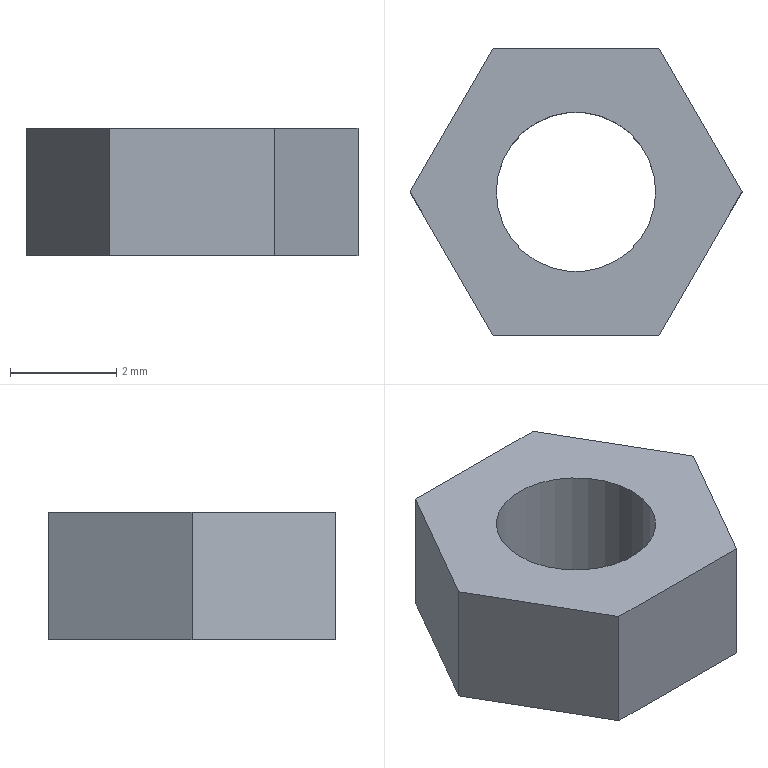Component | NX | NUT | 1 solid | 9 faces | box 6.25 x 5.41 x 2.4 mm | volume 44 mm3 | plane 8 | cylinder 1 | commonest cylinder face diameters 3 x1
STEP:
#1=CARTESIAN_POINT('',(0.,0.,0.));
#2=DIRECTION('',(0.,0.,1.));
#3=DIRECTION('',(1.,0.,0.));
#4=AXIS2_PLACEMENT_3D('',#1,#2,#3);
#5=CARTESIAN_POINT('',(-103.343,127.67,-8.98));
#6=VERTEX_POINT('',#5);
#7=CARTESIAN_POINT('',(-101.781,124.965,-8.98));
#8=VERTEX_POINT('',#7);
#9=CARTESIAN_POINT('',(-103.343,127.67,-8.98));
#10=DIRECTION('',(0.5,-0.866,0.));
#11=VECTOR('',#10,1.);
#12=LINE('',#9,#11);
#13=CARTESIAN_POINT('',(-103.343,127.67,-11.38));
#14=DIRECTION('',(-0.866,-0.5,0.));
#15=DIRECTION('',(0.5,-0.866,0.));
#16=AXIS2_PLACEMENT_3D('',#13,#14,#15);
#17=PLANE('',#16);
#18=CARTESIAN_POINT('',(0.,2.4));
#19=DIRECTION('',(1.,0.));
#20=VECTOR('',#19,1.);
#21=LINE('',#18,#20);
#22=(GEOMETRIC_REPRESENTATION_CONTEXT(2)PARAMETRIC_REPRESENTATION_CONTEXT()REPRESENTATION_CONTEXT('',''));
#23=DEFINITIONAL_REPRESENTATION('',(#21),#22);
#24=PCURVE('',#17,#23);
#25=CARTESIAN_POINT('',(-100.219,127.67,-8.98));
#26=DIRECTION('',(0.,0.,1.));
#27=DIRECTION('',(1.,0.,0.));
#28=AXIS2_PLACEMENT_3D('',#25,#26,#27);
#29=PLANE('',#28);
#30=CARTESIAN_POINT('',(-3.123,0.));
#31=DIRECTION('',(0.5,-0.866));
#32=VECTOR('',#31,1.);
#33=LINE('',#30,#32);
#34=(GEOMETRIC_REPRESENTATION_CONTEXT(2)PARAMETRIC_REPRESENTATION_CONTEXT()REPRESENTATION_CONTEXT('',''));
#35=DEFINITIONAL_REPRESENTATION('',(#33),#34);
#36=PCURVE('',#29,#35);
#37=SURFACE_CURVE('',#12,(#24,#36),.PCURVE_S1.);
#38=EDGE_CURVE('',#6,#8,#37,.T.);
#39=ORIENTED_EDGE('',*,*,#38,.F.);
#40=CARTESIAN_POINT('',(-103.343,127.67,-11.38));
#41=VERTEX_POINT('',#40);
#42=CARTESIAN_POINT('',(-103.343,127.67,-11.38));
#43=DIRECTION('',(0.,0.,1.));
#44=VECTOR('',#43,1.);
#45=LINE('',#42,#44);
#46=CARTESIAN_POINT('',(0.,0.));
#47=DIRECTION('',(0.,1.));
#48=VECTOR('',#47,1.);
#49=LINE('',#46,#48);
#50=(GEOMETRIC_REPRESENTATION_CONTEXT(2)PARAMETRIC_REPRESENTATION_CONTEXT()REPRESENTATION_CONTEXT('',''));
#51=DEFINITIONAL_REPRESENTATION('',(#49),#50);
#52=PCURVE('',#17,#51);
#53=CARTESIAN_POINT('',(-101.781,130.375,-11.38));
#54=DIRECTION('',(-0.866,0.5,0.));
#55=DIRECTION('',(-0.5,-0.866,0.));
#56=AXIS2_PLACEMENT_3D('',#53,#54,#55);
#57=PLANE('',#56);
#58=CARTESIAN_POINT('',(3.123,0.));
#59=DIRECTION('',(0.,1.));
#60=VECTOR('',#59,1.);
#61=LINE('',#58,#60);
#62=(GEOMETRIC_REPRESENTATION_CONTEXT(2)PARAMETRIC_REPRESENTATION_CONTEXT()REPRESENTATION_CONTEXT('',''));
#63=DEFINITIONAL_REPRESENTATION('',(#61),#62);
#64=PCURVE('',#57,#63);
#65=SURFACE_CURVE('',#45,(#52,#64),.PCURVE_S1.);
#66=EDGE_CURVE('',#41,#6,#65,.T.);
#67=ORIENTED_EDGE('',*,*,#66,.F.);
#68=CARTESIAN_POINT('',(-101.781,124.965,-11.38));
#69=VERTEX_POINT('',#68);
#70=CARTESIAN_POINT('',(-103.343,127.67,-11.38));
#71=DIRECTION('',(0.5,-0.866,0.));
#72=VECTOR('',#71,1.);
#73=LINE('',#70,#72);
#74=CARTESIAN_POINT('',(0.,0.));
#75=DIRECTION('',(1.,0.));
#76=VECTOR('',#75,1.);
#77=LINE('',#74,#76);
#78=(GEOMETRIC_REPRESENTATION_CONTEXT(2)PARAMETRIC_REPRESENTATION_CONTEXT()REPRESENTATION_CONTEXT('',''));
#79=DEFINITIONAL_REPRESENTATION('',(#77),#78);
#80=PCURVE('',#17,#79);
#81=CARTESIAN_POINT('',(-100.219,127.67,-11.38));
#82=DIRECTION('',(0.,0.,1.));
#83=DIRECTION('',(1.,0.,0.));
#84=AXIS2_PLACEMENT_3D('',#81,#82,#83);
#85=PLANE('',#84);
#86=CARTESIAN_POINT('',(-3.123,0.));
#87=DIRECTION('',(0.5,-0.866));
#88=VECTOR('',#87,1.);
#89=LINE('',#86,#88);
#90=(GEOMETRIC_REPRESENTATION_CONTEXT(2)PARAMETRIC_REPRESENTATION_CONTEXT()REPRESENTATION_CONTEXT('',''));
#91=DEFINITIONAL_REPRESENTATION('',(#89),#90);
#92=PCURVE('',#85,#91);
#93=SURFACE_CURVE('',#73,(#80,#92),.PCURVE_S1.);
#94=EDGE_CURVE('',#41,#69,#93,.T.);
#95=ORIENTED_EDGE('',*,*,#94,.T.);
#96=CARTESIAN_POINT('',(-101.781,124.965,-11.38));
#97=DIRECTION('',(0.,0.,1.));
#98=VECTOR('',#97,1.);
#99=LINE('',#96,#98);
#100=CARTESIAN_POINT('',(3.123,0.));
#101=DIRECTION('',(0.,1.));
#102=VECTOR('',#101,1.);
#103=LINE('',#100,#102);
#104=(GEOMETRIC_REPRESENTATION_CONTEXT(2)PARAMETRIC_REPRESENTATION_CONTEXT()REPRESENTATION_CONTEXT('',''));
#105=DEFINITIONAL_REPRESENTATION('',(#103),#104);
#106=PCURVE('',#17,#105);
#107=CARTESIAN_POINT('',(-101.781,124.965,-11.38));
#108=DIRECTION('',(-0.,-1.,0.));
#109=DIRECTION('',(1.,-0.,0.));
#110=AXIS2_PLACEMENT_3D('',#107,#108,#109);
#111=PLANE('',#110);
#112=CARTESIAN_POINT('',(0.,0.));
#113=DIRECTION('',(0.,1.));
#114=VECTOR('',#113,1.);
#115=LINE('',#112,#114);
#116=(GEOMETRIC_REPRESENTATION_CONTEXT(2)PARAMETRIC_REPRESENTATION_CONTEXT()REPRESENTATION_CONTEXT('',''));
#117=DEFINITIONAL_REPRESENTATION('',(#115),#116);
#118=PCURVE('',#111,#117);
#119=SURFACE_CURVE('',#99,(#106,#118),.PCURVE_S1.);
#120=EDGE_CURVE('',#69,#8,#119,.T.);
#121=ORIENTED_EDGE('',*,*,#120,.T.);
#122=EDGE_LOOP('',(#39,#67,#95,#121));
#123=FACE_BOUND('',#122,.T.);
#124=ADVANCED_FACE('',(#123),#17,.T.);
#125=CARTESIAN_POINT('',(-98.657,124.965,-8.98));
#126=VERTEX_POINT('',#125);
#127=CARTESIAN_POINT('',(-101.781,124.965,-8.98));
#128=DIRECTION('',(1.,-0.,0.));
#129=VECTOR('',#128,1.);
#130=LINE('',#127,#129);
#131=CARTESIAN_POINT('',(0.,2.4));
#132=DIRECTION('',(1.,0.));
#133=VECTOR('',#132,1.);
#134=LINE('',#131,#133);
#135=(GEOMETRIC_REPRESENTATION_CONTEXT(2)PARAMETRIC_REPRESENTATION_CONTEXT()REPRESENTATION_CONTEXT('',''));
#136=DEFINITIONAL_REPRESENTATION('',(#134),#135);
#137=PCURVE('',#111,#136);
#138=CARTESIAN_POINT('',(-1.562,-2.705));
#139=DIRECTION('',(1.,-0.));
#140=VECTOR('',#139,1.);
#141=LINE('',#138,#140);
#142=(GEOMETRIC_REPRESENTATION_CONTEXT(2)PARAMETRIC_REPRESENTATION_CONTEXT()REPRESENTATION_CONTEXT('',''));
#143=DEFINITIONAL_REPRESENTATION('',(#141),#142);
#144=PCURVE('',#29,#143);
#145=SURFACE_CURVE('',#130,(#137,#144),.PCURVE_S1.);
#146=EDGE_CURVE('',#8,#126,#145,.T.);
#147=ORIENTED_EDGE('',*,*,#146,.F.);
#148=ORIENTED_EDGE('',*,*,#120,.F.);
#149=CARTESIAN_POINT('',(-98.657,124.965,-11.38));
#150=VERTEX_POINT('',#149);
#151=CARTESIAN_POINT('',(-101.781,124.965,-11.38));
#152=DIRECTION('',(1.,-0.,0.));
#153=VECTOR('',#152,1.);
#154=LINE('',#151,#153);
#155=CARTESIAN_POINT('',(0.,0.));
#156=DIRECTION('',(1.,0.));
#157=VECTOR('',#156,1.);
#158=LINE('',#155,#157);
#159=(GEOMETRIC_REPRESENTATION_CONTEXT(2)PARAMETRIC_REPRESENTATION_CONTEXT()REPRESENTATION_CONTEXT('',''));
#160=DEFINITIONAL_REPRESENTATION('',(#158),#159);
#161=PCURVE('',#111,#160);
#162=CARTESIAN_POINT('',(-1.562,-2.705));
#163=DIRECTION('',(1.,-0.));
#164=VECTOR('',#163,1.);
#165=LINE('',#162,#164);
#166=(GEOMETRIC_REPRESENTATION_CONTEXT(2)PARAMETRIC_REPRESENTATION_CONTEXT()REPRESENTATION_CONTEXT('',''));
#167=DEFINITIONAL_REPRESENTATION('',(#165),#166);
#168=PCURVE('',#85,#167);
#169=SURFACE_CURVE('',#154,(#161,#168),.PCURVE_S1.);
#170=EDGE_CURVE('',#69,#150,#169,.T.);
#171=ORIENTED_EDGE('',*,*,#170,.T.);
#172=CARTESIAN_POINT('',(-98.657,124.965,-11.38));
#173=DIRECTION('',(0.,0.,1.));
#174=VECTOR('',#173,1.);
#175=LINE('',#172,#174);
#176=CARTESIAN_POINT('',(3.123,0.));
#177=DIRECTION('',(0.,1.));
#178=VECTOR('',#177,1.);
#179=LINE('',#176,#178);
#180=(GEOMETRIC_REPRESENTATION_CONTEXT(2)PARAMETRIC_REPRESENTATION_CONTEXT()REPRESENTATION_CONTEXT('',''));
#181=DEFINITIONAL_REPRESENTATION('',(#179),#180);
#182=PCURVE('',#111,#181);
#183=CARTESIAN_POINT('',(-98.657,124.965,-11.38));
#184=DIRECTION('',(0.866,-0.5,0.));
#185=DIRECTION('',(0.5,0.866,0.));
#186=AXIS2_PLACEMENT_3D('',#183,#184,#185);
#187=PLANE('',#186);
#188=CARTESIAN_POINT('',(0.,0.));
#189=DIRECTION('',(0.,1.));
#190=VECTOR('',#189,1.);
#191=LINE('',#188,#190);
#192=(GEOMETRIC_REPRESENTATION_CONTEXT(2)PARAMETRIC_REPRESENTATION_CONTEXT()REPRESENTATION_CONTEXT('',''));
#193=DEFINITIONAL_REPRESENTATION('',(#191),#192);
#194=PCURVE('',#187,#193);
#195=SURFACE_CURVE('',#175,(#182,#194),.PCURVE_S1.);
#196=EDGE_CURVE('',#150,#126,#195,.T.);
#197=ORIENTED_EDGE('',*,*,#196,.T.);
#198=EDGE_LOOP('',(#147,#148,#171,#197));
#199=FACE_BOUND('',#198,.T.);
#200=ADVANCED_FACE('',(#199),#111,.T.);
#201=CARTESIAN_POINT('',(-97.096,127.67,-8.98));
#202=VERTEX_POINT('',#201);
#203=CARTESIAN_POINT('',(-98.657,124.965,-8.98));
#204=DIRECTION('',(0.5,0.866,0.));
#205=VECTOR('',#204,1.);
#206=LINE('',#203,#205);
#207=CARTESIAN_POINT('',(0.,2.4));
#208=DIRECTION('',(1.,0.));
#209=VECTOR('',#208,1.);
#210=LINE('',#207,#209);
#211=(GEOMETRIC_REPRESENTATION_CONTEXT(2)PARAMETRIC_REPRESENTATION_CONTEXT()REPRESENTATION_CONTEXT('',''));
#212=DEFINITIONAL_REPRESENTATION('',(#210),#211);
#213=PCURVE('',#187,#212);
#214=CARTESIAN_POINT('',(1.562,-2.705));
#215=DIRECTION('',(0.5,0.866));
#216=VECTOR('',#215,1.);
#217=LINE('',#214,#216);
#218=(GEOMETRIC_REPRESENTATION_CONTEXT(2)PARAMETRIC_REPRESENTATION_CONTEXT()REPRESENTATION_CONTEXT('',''));
#219=DEFINITIONAL_REPRESENTATION('',(#217),#218);
#220=PCURVE('',#29,#219);
#221=SURFACE_CURVE('',#206,(#213,#220),.PCURVE_S1.);
#222=EDGE_CURVE('',#126,#202,#221,.T.);
#223=ORIENTED_EDGE('',*,*,#222,.F.);
#224=ORIENTED_EDGE('',*,*,#196,.F.);
#225=CARTESIAN_POINT('',(-97.096,127.67,-11.38));
#226=VERTEX_POINT('',#225);
#227=CARTESIAN_POINT('',(-98.657,124.965,-11.38));
#228=DIRECTION('',(0.5,0.866,0.));
#229=VECTOR('',#228,1.);
#230=LINE('',#227,#229);
#231=CARTESIAN_POINT('',(0.,0.));
#232=DIRECTION('',(1.,0.));
#233=VECTOR('',#232,1.);
#234=LINE('',#231,#233);
#235=(GEOMETRIC_REPRESENTATION_CONTEXT(2)PARAMETRIC_REPRESENTATION_CONTEXT()REPRESENTATION_CONTEXT('',''));
#236=DEFINITIONAL_REPRESENTATION('',(#234),#235);
#237=PCURVE('',#187,#236);
#238=CARTESIAN_POINT('',(1.562,-2.705));
#239=DIRECTION('',(0.5,0.866));
#240=VECTOR('',#239,1.);
#241=LINE('',#238,#240);
#242=(GEOMETRIC_REPRESENTATION_CONTEXT(2)PARAMETRIC_REPRESENTATION_CONTEXT()REPRESENTATION_CONTEXT('',''));
#243=DEFINITIONAL_REPRESENTATION('',(#241),#242);
#244=PCURVE('',#85,#243);
#245=SURFACE_CURVE('',#230,(#237,#244),.PCURVE_S1.);
#246=EDGE_CURVE('',#150,#226,#245,.T.);
#247=ORIENTED_EDGE('',*,*,#246,.T.);
#248=CARTESIAN_POINT('',(-97.096,127.67,-11.38));
#249=DIRECTION('',(0.,0.,1.));
#250=VECTOR('',#249,1.);
#251=LINE('',#248,#250);
#252=CARTESIAN_POINT('',(3.123,0.));
#253=DIRECTION('',(0.,1.));
#254=VECTOR('',#253,1.);
#255=LINE('',#252,#254);
#256=(GEOMETRIC_REPRESENTATION_CONTEXT(2)PARAMETRIC_REPRESENTATION_CONTEXT()REPRESENTATION_CONTEXT('',''));
#257=DEFINITIONAL_REPRESENTATION('',(#255),#256);
#258=PCURVE('',#187,#257);
#259=CARTESIAN_POINT('',(-97.096,127.67,-11.38));
#260=DIRECTION('',(0.866,0.5,0.));
#261=DIRECTION('',(-0.5,0.866,0.));
#262=AXIS2_PLACEMENT_3D('',#259,#260,#261);
#263=PLANE('',#262);
#264=CARTESIAN_POINT('',(0.,0.));
#265=DIRECTION('',(0.,1.));
#266=VECTOR('',#265,1.);
#267=LINE('',#264,#266);
#268=(GEOMETRIC_REPRESENTATION_CONTEXT(2)PARAMETRIC_REPRESENTATION_CONTEXT()REPRESENTATION_CONTEXT('',''));
#269=DEFINITIONAL_REPRESENTATION('',(#267),#268);
#270=PCURVE('',#263,#269);
#271=SURFACE_CURVE('',#251,(#258,#270),.PCURVE_S1.);
#272=EDGE_CURVE('',#226,#202,#271,.T.);
#273=ORIENTED_EDGE('',*,*,#272,.T.);
#274=EDGE_LOOP('',(#223,#224,#247,#273));
#275=FACE_BOUND('',#274,.T.);
#276=ADVANCED_FACE('',(#275),#187,.T.);
#277=CARTESIAN_POINT('',(-98.657,130.375,-8.98));
#278=VERTEX_POINT('',#277);
#279=CARTESIAN_POINT('',(-97.096,127.67,-8.98));
#280=DIRECTION('',(-0.5,0.866,0.));
#281=VECTOR('',#280,1.);
#282=LINE('',#279,#281);
#283=CARTESIAN_POINT('',(0.,2.4));
#284=DIRECTION('',(1.,0.));
#285=VECTOR('',#284,1.);
#286=LINE('',#283,#285);
#287=(GEOMETRIC_REPRESENTATION_CONTEXT(2)PARAMETRIC_REPRESENTATION_CONTEXT()REPRESENTATION_CONTEXT('',''));
#288=DEFINITIONAL_REPRESENTATION('',(#286),#287);
#289=PCURVE('',#263,#288);
#290=CARTESIAN_POINT('',(3.123,0.));
#291=DIRECTION('',(-0.5,0.866));
#292=VECTOR('',#291,1.);
#293=LINE('',#290,#292);
#294=(GEOMETRIC_REPRESENTATION_CONTEXT(2)PARAMETRIC_REPRESENTATION_CONTEXT()REPRESENTATION_CONTEXT('',''));
#295=DEFINITIONAL_REPRESENTATION('',(#293),#294);
#296=PCURVE('',#29,#295);
#297=SURFACE_CURVE('',#282,(#289,#296),.PCURVE_S1.);
#298=EDGE_CURVE('',#202,#278,#297,.T.);
#299=ORIENTED_EDGE('',*,*,#298,.F.);
#300=ORIENTED_EDGE('',*,*,#272,.F.);
#301=CARTESIAN_POINT('',(-98.657,130.375,-11.38));
#302=VERTEX_POINT('',#301);
#303=CARTESIAN_POINT('',(-97.096,127.67,-11.38));
#304=DIRECTION('',(-0.5,0.866,0.));
#305=VECTOR('',#304,1.);
#306=LINE('',#303,#305);
#307=CARTESIAN_POINT('',(0.,0.));
#308=DIRECTION('',(1.,0.));
#309=VECTOR('',#308,1.);
#310=LINE('',#307,#309);
#311=(GEOMETRIC_REPRESENTATION_CONTEXT(2)PARAMETRIC_REPRESENTATION_CONTEXT()REPRESENTATION_CONTEXT('',''));
#312=DEFINITIONAL_REPRESENTATION('',(#310),#311);
#313=PCURVE('',#263,#312);
#314=CARTESIAN_POINT('',(3.123,0.));
#315=DIRECTION('',(-0.5,0.866));
#316=VECTOR('',#315,1.);
#317=LINE('',#314,#316);
#318=(GEOMETRIC_REPRESENTATION_CONTEXT(2)PARAMETRIC_REPRESENTATION_CONTEXT()REPRESENTATION_CONTEXT('',''));
#319=DEFINITIONAL_REPRESENTATION('',(#317),#318);
#320=PCURVE('',#85,#319);
#321=SURFACE_CURVE('',#306,(#313,#320),.PCURVE_S1.);
#322=EDGE_CURVE('',#226,#302,#321,.T.);
#323=ORIENTED_EDGE('',*,*,#322,.T.);
#324=CARTESIAN_POINT('',(-98.657,130.375,-11.38));
#325=DIRECTION('',(0.,0.,1.));
#326=VECTOR('',#325,1.);
#327=LINE('',#324,#326);
#328=CARTESIAN_POINT('',(3.123,0.));
#329=DIRECTION('',(0.,1.));
#330=VECTOR('',#329,1.);
#331=LINE('',#328,#330);
#332=(GEOMETRIC_REPRESENTATION_CONTEXT(2)PARAMETRIC_REPRESENTATION_CONTEXT()REPRESENTATION_CONTEXT('',''));
#333=DEFINITIONAL_REPRESENTATION('',(#331),#332);
#334=PCURVE('',#263,#333);
#335=CARTESIAN_POINT('',(-98.657,130.375,-11.38));
#336=DIRECTION('',(0.,1.,0.));
#337=DIRECTION('',(-1.,0.,0.));
#338=AXIS2_PLACEMENT_3D('',#335,#336,#337);
#339=PLANE('',#338);
#340=CARTESIAN_POINT('',(0.,0.));
#341=DIRECTION('',(0.,1.));
#342=VECTOR('',#341,1.);
#343=LINE('',#340,#342);
#344=(GEOMETRIC_REPRESENTATION_CONTEXT(2)PARAMETRIC_REPRESENTATION_CONTEXT()REPRESENTATION_CONTEXT('',''));
#345=DEFINITIONAL_REPRESENTATION('',(#343),#344);
#346=PCURVE('',#339,#345);
#347=SURFACE_CURVE('',#327,(#334,#346),.PCURVE_S1.);
#348=EDGE_CURVE('',#302,#278,#347,.T.);
#349=ORIENTED_EDGE('',*,*,#348,.T.);
#350=EDGE_LOOP('',(#299,#300,#323,#349));
#351=FACE_BOUND('',#350,.T.);
#352=ADVANCED_FACE('',(#351),#263,.T.);
#353=CARTESIAN_POINT('',(-101.781,130.375,-8.98));
#354=VERTEX_POINT('',#353);
#355=CARTESIAN_POINT('',(-98.657,130.375,-8.98));
#356=DIRECTION('',(-1.,0.,0.));
#357=VECTOR('',#356,1.);
#358=LINE('',#355,#357);
#359=CARTESIAN_POINT('',(0.,2.4));
#360=DIRECTION('',(1.,0.));
#361=VECTOR('',#360,1.);
#362=LINE('',#359,#361);
#363=(GEOMETRIC_REPRESENTATION_CONTEXT(2)PARAMETRIC_REPRESENTATION_CONTEXT()REPRESENTATION_CONTEXT('',''));
#364=DEFINITIONAL_REPRESENTATION('',(#362),#363);
#365=PCURVE('',#339,#364);
#366=CARTESIAN_POINT('',(1.562,2.705));
#367=DIRECTION('',(-1.,0.));
#368=VECTOR('',#367,1.);
#369=LINE('',#366,#368);
#370=(GEOMETRIC_REPRESENTATION_CONTEXT(2)PARAMETRIC_REPRESENTATION_CONTEXT()REPRESENTATION_CONTEXT('',''));
#371=DEFINITIONAL_REPRESENTATION('',(#369),#370);
#372=PCURVE('',#29,#371);
#373=SURFACE_CURVE('',#358,(#365,#372),.PCURVE_S1.);
#374=EDGE_CURVE('',#278,#354,#373,.T.);
#375=ORIENTED_EDGE('',*,*,#374,.F.);
#376=ORIENTED_EDGE('',*,*,#348,.F.);
#377=CARTESIAN_POINT('',(-101.781,130.375,-11.38));
#378=VERTEX_POINT('',#377);
#379=CARTESIAN_POINT('',(-98.657,130.375,-11.38));
#380=DIRECTION('',(-1.,0.,0.));
#381=VECTOR('',#380,1.);
#382=LINE('',#379,#381);
#383=CARTESIAN_POINT('',(0.,0.));
#384=DIRECTION('',(1.,0.));
#385=VECTOR('',#384,1.);
#386=LINE('',#383,#385);
#387=(GEOMETRIC_REPRESENTATION_CONTEXT(2)PARAMETRIC_REPRESENTATION_CONTEXT()REPRESENTATION_CONTEXT('',''));
#388=DEFINITIONAL_REPRESENTATION('',(#386),#387);
#389=PCURVE('',#339,#388);
#390=CARTESIAN_POINT('',(1.562,2.705));
#391=DIRECTION('',(-1.,0.));
#392=VECTOR('',#391,1.);
#393=LINE('',#390,#392);
#394=(GEOMETRIC_REPRESENTATION_CONTEXT(2)PARAMETRIC_REPRESENTATION_CONTEXT()REPRESENTATION_CONTEXT('',''));
#395=DEFINITIONAL_REPRESENTATION('',(#393),#394);
#396=PCURVE('',#85,#395);
#397=SURFACE_CURVE('',#382,(#389,#396),.PCURVE_S1.);
#398=EDGE_CURVE('',#302,#378,#397,.T.);
#399=ORIENTED_EDGE('',*,*,#398,.T.);
#400=CARTESIAN_POINT('',(-101.781,130.375,-11.38));
#401=DIRECTION('',(0.,0.,1.));
#402=VECTOR('',#401,1.);
#403=LINE('',#400,#402);
#404=CARTESIAN_POINT('',(3.123,0.));
#405=DIRECTION('',(0.,1.));
#406=VECTOR('',#405,1.);
#407=LINE('',#404,#406);
#408=(GEOMETRIC_REPRESENTATION_CONTEXT(2)PARAMETRIC_REPRESENTATION_CONTEXT()REPRESENTATION_CONTEXT('',''));
#409=DEFINITIONAL_REPRESENTATION('',(#407),#408);
#410=PCURVE('',#339,#409);
#411=CARTESIAN_POINT('',(0.,0.));
#412=DIRECTION('',(0.,1.));
#413=VECTOR('',#412,1.);
#414=LINE('',#411,#413);
#415=(GEOMETRIC_REPRESENTATION_CONTEXT(2)PARAMETRIC_REPRESENTATION_CONTEXT()REPRESENTATION_CONTEXT('',''));
#416=DEFINITIONAL_REPRESENTATION('',(#414),#415);
#417=PCURVE('',#57,#416);
#418=SURFACE_CURVE('',#403,(#410,#417),.PCURVE_S1.);
#419=EDGE_CURVE('',#378,#354,#418,.T.);
#420=ORIENTED_EDGE('',*,*,#419,.T.);
#421=EDGE_LOOP('',(#375,#376,#399,#420));
#422=FACE_BOUND('',#421,.T.);
#423=ADVANCED_FACE('',(#422),#339,.T.);
#424=CARTESIAN_POINT('',(-101.781,130.375,-8.98));
#425=DIRECTION('',(-0.5,-0.866,0.));
#426=VECTOR('',#425,1.);
#427=LINE('',#424,#426);
#428=CARTESIAN_POINT('',(0.,2.4));
#429=DIRECTION('',(1.,0.));
#430=VECTOR('',#429,1.);
#431=LINE('',#428,#430);
#432=(GEOMETRIC_REPRESENTATION_CONTEXT(2)PARAMETRIC_REPRESENTATION_CONTEXT()REPRESENTATION_CONTEXT('',''));
#433=DEFINITIONAL_REPRESENTATION('',(#431),#432);
#434=PCURVE('',#57,#433);
#435=CARTESIAN_POINT('',(-1.562,2.705));
#436=DIRECTION('',(-0.5,-0.866));
#437=VECTOR('',#436,1.);
#438=LINE('',#435,#437);
#439=(GEOMETRIC_REPRESENTATION_CONTEXT(2)PARAMETRIC_REPRESENTATION_CONTEXT()REPRESENTATION_CONTEXT('',''));
#440=DEFINITIONAL_REPRESENTATION('',(#438),#439);
#441=PCURVE('',#29,#440);
#442=SURFACE_CURVE('',#427,(#434,#441),.PCURVE_S1.);
#443=EDGE_CURVE('',#354,#6,#442,.T.);
#444=ORIENTED_EDGE('',*,*,#443,.F.);
#445=ORIENTED_EDGE('',*,*,#419,.F.);
#446=CARTESIAN_POINT('',(-101.781,130.375,-11.38));
#447=DIRECTION('',(-0.5,-0.866,0.));
#448=VECTOR('',#447,1.);
#449=LINE('',#446,#448);
#450=CARTESIAN_POINT('',(0.,0.));
#451=DIRECTION('',(1.,0.));
#452=VECTOR('',#451,1.);
#453=LINE('',#450,#452);
#454=(GEOMETRIC_REPRESENTATION_CONTEXT(2)PARAMETRIC_REPRESENTATION_CONTEXT()REPRESENTATION_CONTEXT('',''));
#455=DEFINITIONAL_REPRESENTATION('',(#453),#454);
#456=PCURVE('',#57,#455);
#457=CARTESIAN_POINT('',(-1.562,2.705));
#458=DIRECTION('',(-0.5,-0.866));
#459=VECTOR('',#458,1.);
#460=LINE('',#457,#459);
#461=(GEOMETRIC_REPRESENTATION_CONTEXT(2)PARAMETRIC_REPRESENTATION_CONTEXT()REPRESENTATION_CONTEXT('',''));
#462=DEFINITIONAL_REPRESENTATION('',(#460),#461);
#463=PCURVE('',#85,#462);
#464=SURFACE_CURVE('',#449,(#456,#463),.PCURVE_S1.);
#465=EDGE_CURVE('',#378,#41,#464,.T.);
#466=ORIENTED_EDGE('',*,*,#465,.T.);
#467=ORIENTED_EDGE('',*,*,#66,.T.);
#468=EDGE_LOOP('',(#444,#445,#466,#467));
#469=FACE_BOUND('',#468,.T.);
#470=ADVANCED_FACE('',(#469),#57,.T.);
#471=CARTESIAN_POINT('',(-98.719,127.67,-11.38));
#472=VERTEX_POINT('',#471);
#473=CARTESIAN_POINT('',(-100.219,127.67,-11.38));
#474=DIRECTION('',(0.,0.,1.));
#475=DIRECTION('',(1.,0.,0.));
#476=AXIS2_PLACEMENT_3D('',#473,#474,#475);
#477=CIRCLE('',#476,1.5);
#478=CARTESIAN_POINT('',(0.,0.));
#479=DIRECTION('',(1.,0.));
#480=AXIS2_PLACEMENT_2D('',#478,#479);
#481=CIRCLE('',#480,1.5);
#482=(GEOMETRIC_REPRESENTATION_CONTEXT(2)PARAMETRIC_REPRESENTATION_CONTEXT()REPRESENTATION_CONTEXT('',''));
#483=DEFINITIONAL_REPRESENTATION('',(#481),#482);
#484=PCURVE('',#85,#483);
#485=CARTESIAN_POINT('',(-100.219,127.67,-12.48));
#486=DIRECTION('',(0.,0.,1.));
#487=DIRECTION('',(1.,0.,0.));
#488=AXIS2_PLACEMENT_3D('',#485,#486,#487);
#489=CYLINDRICAL_SURFACE('',#488,1.5);
#490=CARTESIAN_POINT('',(0.,1.1));
#491=DIRECTION('',(1.,0.));
#492=VECTOR('',#491,1.);
#493=LINE('',#490,#492);
#494=(GEOMETRIC_REPRESENTATION_CONTEXT(2)PARAMETRIC_REPRESENTATION_CONTEXT()REPRESENTATION_CONTEXT('',''));
#495=DEFINITIONAL_REPRESENTATION('',(#493),#494);
#496=PCURVE('',#489,#495);
#497=SURFACE_CURVE('',#477,(#484,#496),.PCURVE_S1.);
#498=EDGE_CURVE('',#472,#472,#497,.T.);
#499=ORIENTED_EDGE('',*,*,#498,.T.);
#500=EDGE_LOOP('',(#499));
#501=FACE_BOUND('',#500,.T.);
#502=ORIENTED_EDGE('',*,*,#94,.F.);
#503=ORIENTED_EDGE('',*,*,#465,.F.);
#504=ORIENTED_EDGE('',*,*,#398,.F.);
#505=ORIENTED_EDGE('',*,*,#322,.F.);
#506=ORIENTED_EDGE('',*,*,#246,.F.);
#507=ORIENTED_EDGE('',*,*,#170,.F.);
#508=EDGE_LOOP('',(#502,#503,#504,#505,#506,#507));
#509=FACE_BOUND('',#508,.T.);
#510=ADVANCED_FACE('',(#501,#509),#85,.F.);
#511=CARTESIAN_POINT('',(-98.719,127.67,-8.98));
#512=VERTEX_POINT('',#511);
#513=CARTESIAN_POINT('',(-100.219,127.67,-8.98));
#514=DIRECTION('',(0.,0.,1.));
#515=DIRECTION('',(1.,0.,0.));
#516=AXIS2_PLACEMENT_3D('',#513,#514,#515);
#517=CIRCLE('',#516,1.5);
#518=CARTESIAN_POINT('',(0.,0.));
#519=DIRECTION('',(1.,0.));
#520=AXIS2_PLACEMENT_2D('',#518,#519);
#521=CIRCLE('',#520,1.5);
#522=(GEOMETRIC_REPRESENTATION_CONTEXT(2)PARAMETRIC_REPRESENTATION_CONTEXT()REPRESENTATION_CONTEXT('',''));
#523=DEFINITIONAL_REPRESENTATION('',(#521),#522);
#524=PCURVE('',#29,#523);
#525=CARTESIAN_POINT('',(0.,3.5));
#526=DIRECTION('',(1.,0.));
#527=VECTOR('',#526,1.);
#528=LINE('',#525,#527);
#529=(GEOMETRIC_REPRESENTATION_CONTEXT(2)PARAMETRIC_REPRESENTATION_CONTEXT()REPRESENTATION_CONTEXT('',''));
#530=DEFINITIONAL_REPRESENTATION('',(#528),#529);
#531=PCURVE('',#489,#530);
#532=SURFACE_CURVE('',#517,(#524,#531),.PCURVE_S1.);
#533=EDGE_CURVE('',#512,#512,#532,.T.);
#534=ORIENTED_EDGE('',*,*,#533,.F.);
#535=EDGE_LOOP('',(#534));
#536=FACE_BOUND('',#535,.T.);
#537=ORIENTED_EDGE('',*,*,#38,.T.);
#538=ORIENTED_EDGE('',*,*,#146,.T.);
#539=ORIENTED_EDGE('',*,*,#222,.T.);
#540=ORIENTED_EDGE('',*,*,#298,.T.);
#541=ORIENTED_EDGE('',*,*,#374,.T.);
#542=ORIENTED_EDGE('',*,*,#443,.T.);
#543=EDGE_LOOP('',(#537,#538,#539,#540,#541,#542));
#544=FACE_BOUND('',#543,.T.);
#545=ADVANCED_FACE('',(#536,#544),#29,.T.);
#546=ORIENTED_EDGE('',*,*,#533,.F.);
#547=CARTESIAN_POINT('',(-98.719,127.67,-11.38));
#548=CARTESIAN_POINT('',(-98.719,127.67,-8.98));
#549=B_SPLINE_CURVE_WITH_KNOTS('',1,(#547,#548),.UNSPECIFIED.,.F.,.F.,(2,2),(1.1,3.5),.PIECEWISE_BEZIER_KNOTS.);
#550=CARTESIAN_POINT('',(0.,0.));
#551=DIRECTION('',(0.,1.));
#552=VECTOR('',#551,1.);
#553=LINE('',#550,#552);
#554=(GEOMETRIC_REPRESENTATION_CONTEXT(2)PARAMETRIC_REPRESENTATION_CONTEXT()REPRESENTATION_CONTEXT('',''));
#555=DEFINITIONAL_REPRESENTATION('',(#553),#554);
#556=PCURVE('',#489,#555);
#557=CARTESIAN_POINT('',(6.283,0.));
#558=DIRECTION('',(0.,1.));
#559=VECTOR('',#558,1.);
#560=LINE('',#557,#559);
#561=(GEOMETRIC_REPRESENTATION_CONTEXT(2)PARAMETRIC_REPRESENTATION_CONTEXT()REPRESENTATION_CONTEXT('',''));
#562=DEFINITIONAL_REPRESENTATION('',(#560),#561);
#563=PCURVE('',#489,#562);
#564=SEAM_CURVE('',#549,(#556,#563),.PCURVE_S1.);
#565=EDGE_CURVE('',#472,#512,#564,.T.);
#566=ORIENTED_EDGE('',*,*,#565,.F.);
#567=ORIENTED_EDGE('',*,*,#498,.T.);
#568=ORIENTED_EDGE('',*,*,#565,.T.);
#569=EDGE_LOOP('',(#546,#566,#567,#568));
#570=FACE_BOUND('',#569,.F.);
#571=ADVANCED_FACE('',(#570),#489,.F.);
#572=CLOSED_SHELL('',(#124,#200,#276,#352,#423,#470,#510,#545,#571));
#573=MANIFOLD_SOLID_BREP('',#572);
#574=(LENGTH_UNIT()NAMED_UNIT(*)SI_UNIT(.MILLI.,.METRE.));
#575=UNCERTAINTY_MEASURE_WITH_UNIT(LENGTH_MEASURE(0.000001),#574,'','');
#576=(NAMED_UNIT(*)PLANE_ANGLE_UNIT()SI_UNIT($,.RADIAN.));
#577=(NAMED_UNIT(*)SI_UNIT($,.STERADIAN.)SOLID_ANGLE_UNIT());
#578=(GEOMETRIC_REPRESENTATION_CONTEXT(3)GLOBAL_UNCERTAINTY_ASSIGNED_CONTEXT((#575))GLOBAL_UNIT_ASSIGNED_CONTEXT((#574,#576,#577))REPRESENTATION_CONTEXT('',''));
#579=ADVANCED_BREP_SHAPE_REPRESENTATION('',(#4,#573),#578);